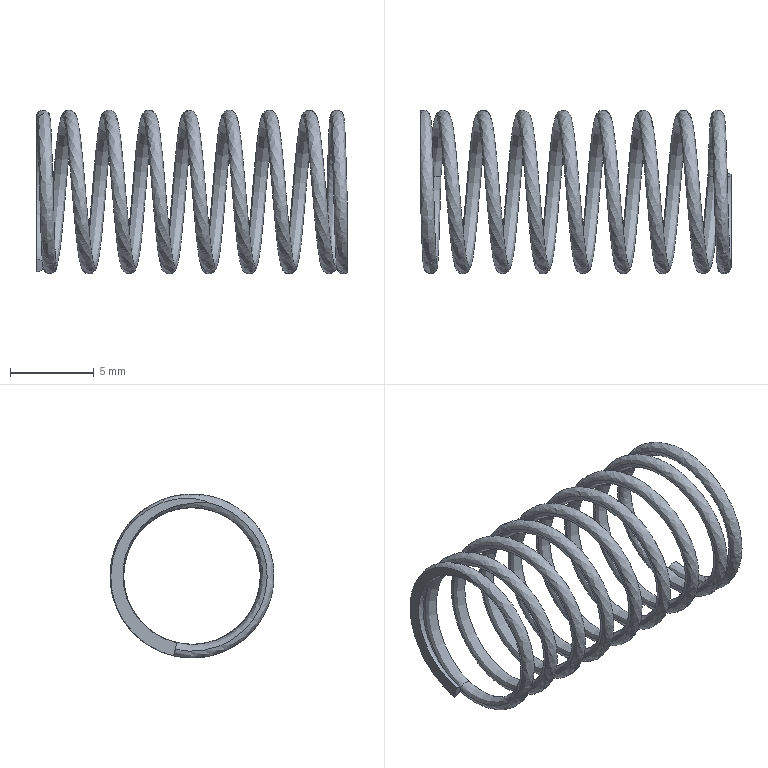Component | SolidWorks | OuterBagSealingSpring-1 | 1 solid | 10 faces | volume 126 mm3 | spline 6 | plane 4